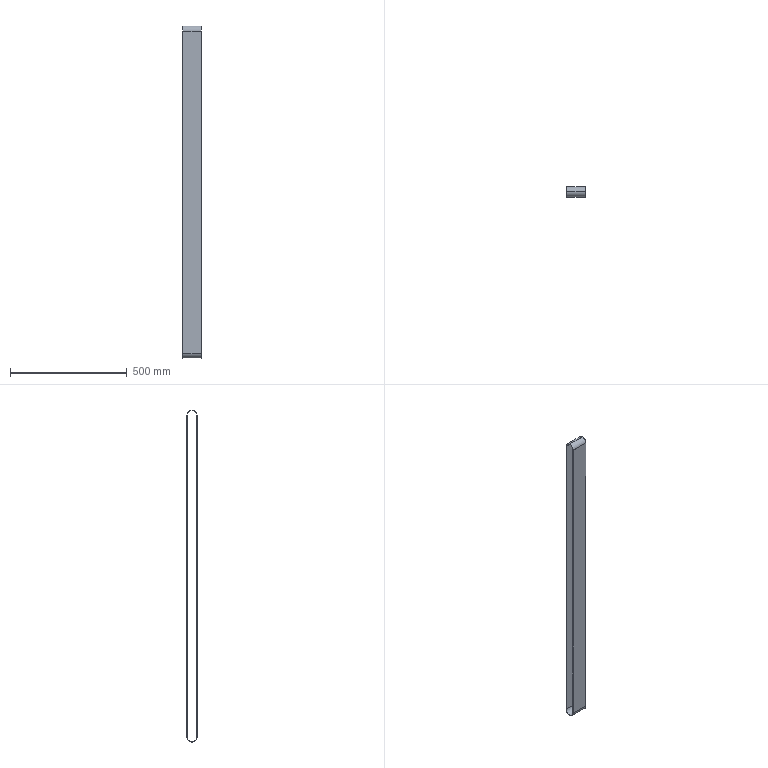Component | SolidWorks | ConveyorBelt-1 | 1 solid | 12 faces | box 78 x 43 x 1423 mm | volume 225572 mm3 | cylinder 6 | plane 6 | commonest cylinder face diameters 41 x3 43 x3
build123d program:
from build123d import *

# Parameters (mm, degrees)
BOSS_EXTRUDE1_DEPTH = 78


with BuildPart() as part:
    # Sketch1 → Boss-Extrude1 (new body)
    with BuildSketch(Plane(origin=(0, 0, 0), x_dir=(0, 0, -1), z_dir=(1, 0, 0))):
        with BuildLine():
            Line((-57.814, 21.5), (1322.186, 21.5))
            ThreePointArc((1322.186, 21.5), (1343.686, 0), (1322.186, -21.5))
            Line((1322.186, -21.5), (-57.814, -21.5))
            ThreePointArc((-57.814, -21.5), (-79.314, 0), (-57.814, 21.5))
        make_face()
        with BuildLine():
            Line((-57.814, 20.5), (1322.186, 20.5))
            ThreePointArc((1322.186, 20.5), (1342.686, 0), (1322.186, -20.5))
            Line((1322.186, -20.5), (-57.814, -20.5))
            ThreePointArc((-57.814, -20.5), (-78.314, 0), (-57.814, 20.5))
        make_face(mode=Mode.SUBTRACT)
    extrude(amount=BOSS_EXTRUDE1_DEPTH)


solid = part.part

# Placed as in the assembly
solid = solid.moved(Location((-44.55, 5.646, 1477.186), (0, 0, 0)))
STEP:
#1=COLOUR_RGB('',0.7922,0.8196,0.9333);
#2=FILL_AREA_STYLE_COLOUR('',#1);
#3=FILL_AREA_STYLE('',(#2));
#4=SURFACE_STYLE_FILL_AREA(#3);
#5=SURFACE_SIDE_STYLE('',(#4));
#6=SURFACE_STYLE_USAGE(.BOTH.,#5);
#7=PRESENTATION_STYLE_ASSIGNMENT((#6));
#8=CARTESIAN_POINT('',(1.317,1.029,60.433));
#9=VERTEX_POINT('',#8);
#10=CARTESIAN_POINT('',(1.317,0.2223,61.24));
#11=VERTEX_POINT('',#10);
#12=CARTESIAN_POINT('',(1.317,0.2223,60.433));
#13=DIRECTION('',(1.,0.,0.));
#14=DIRECTION('',(0.,0.,-1.));
#15=AXIS2_PLACEMENT_3D('',#12,#13,#14);
#16=CIRCLE('',#15,0.8071);
#17=EDGE_CURVE('',#9,#11,#16,.T.);
#18=ORIENTED_EDGE('',*,*,#17,.T.);
#19=CARTESIAN_POINT('',(-1.754,0.2223,61.24));
#20=VERTEX_POINT('',#19);
#21=CARTESIAN_POINT('',(1.317,0.2223,61.24));
#22=DIRECTION('',(-1.,0.,0.));
#23=VECTOR('',#22,39.37);
#24=LINE('',#21,#23);
#25=EDGE_CURVE('',#11,#20,#24,.T.);
#26=ORIENTED_EDGE('',*,*,#25,.T.);
#27=CARTESIAN_POINT('',(-1.754,1.029,60.433));
#28=VERTEX_POINT('',#27);
#29=CARTESIAN_POINT('',(-1.754,0.2223,60.433));
#30=DIRECTION('',(1.,0.,0.));
#31=DIRECTION('',(0.,0.,-1.));
#32=AXIS2_PLACEMENT_3D('',#29,#30,#31);
#33=CIRCLE('',#32,0.8071);
#34=EDGE_CURVE('',#28,#20,#33,.T.);
#35=ORIENTED_EDGE('',*,*,#34,.F.);
#36=CARTESIAN_POINT('',(1.317,1.029,60.433));
#37=DIRECTION('',(-1.,0.,0.));
#38=VECTOR('',#37,39.37);
#39=LINE('',#36,#38);
#40=EDGE_CURVE('',#9,#28,#39,.T.);
#41=ORIENTED_EDGE('',*,*,#40,.F.);
#42=EDGE_LOOP('',(#18,#26,#35,#41));
#43=FACE_OUTER_BOUND('',#42,.T.);
#44=CARTESIAN_POINT('',(1.317,0.2223,60.433));
#45=DIRECTION('',(-1.,0.,0.));
#46=DIRECTION('',(0.,0.,1.));
#47=AXIS2_PLACEMENT_3D('',#44,#45,#46);
#48=CYLINDRICAL_SURFACE('',#47,0.8071);
#49=ADVANCED_FACE('',(#43),#48,.F.);
#50=CARTESIAN_POINT('',(1.317,0.2223,61.28));
#51=VERTEX_POINT('',#50);
#52=CARTESIAN_POINT('',(1.317,-0.6242,60.433));
#53=VERTEX_POINT('',#52);
#54=CARTESIAN_POINT('',(1.317,0.2223,60.433));
#55=DIRECTION('',(1.,0.,0.));
#56=DIRECTION('',(0.,0.,-1.));
#57=AXIS2_PLACEMENT_3D('',#54,#55,#56);
#58=CIRCLE('',#57,0.8465);
#59=EDGE_CURVE('',#51,#53,#58,.T.);
#60=ORIENTED_EDGE('',*,*,#59,.F.);
#61=CARTESIAN_POINT('',(-1.754,0.2223,61.28));
#62=VERTEX_POINT('',#61);
#63=CARTESIAN_POINT('',(1.317,0.2223,61.28));
#64=DIRECTION('',(-1.,0.,0.));
#65=VECTOR('',#64,39.37);
#66=LINE('',#63,#65);
#67=EDGE_CURVE('',#51,#62,#66,.T.);
#68=ORIENTED_EDGE('',*,*,#67,.T.);
#69=CARTESIAN_POINT('',(-1.754,-0.6242,60.433));
#70=VERTEX_POINT('',#69);
#71=CARTESIAN_POINT('',(-1.754,0.2223,60.433));
#72=DIRECTION('',(1.,0.,0.));
#73=DIRECTION('',(0.,0.,-1.));
#74=AXIS2_PLACEMENT_3D('',#71,#72,#73);
#75=CIRCLE('',#74,0.8465);
#76=EDGE_CURVE('',#62,#70,#75,.T.);
#77=ORIENTED_EDGE('',*,*,#76,.T.);
#78=CARTESIAN_POINT('',(1.317,-0.6242,60.433));
#79=DIRECTION('',(-1.,0.,0.));
#80=VECTOR('',#79,39.37);
#81=LINE('',#78,#80);
#82=EDGE_CURVE('',#53,#70,#81,.T.);
#83=ORIENTED_EDGE('',*,*,#82,.F.);
#84=EDGE_LOOP('',(#60,#68,#77,#83));
#85=FACE_OUTER_BOUND('',#84,.T.);
#86=CARTESIAN_POINT('',(1.317,0.2223,60.433));
#87=DIRECTION('',(-1.,0.,0.));
#88=DIRECTION('',(0.,0.,1.));
#89=AXIS2_PLACEMENT_3D('',#86,#87,#88);
#90=CYLINDRICAL_SURFACE('',#89,0.8465);
#91=ADVANCED_FACE('',(#85),#90,.T.);
#92=CARTESIAN_POINT('',(1.317,1.069,60.433));
#93=VERTEX_POINT('',#92);
#94=CARTESIAN_POINT('',(1.317,0.2223,60.433));
#95=DIRECTION('',(1.,0.,0.));
#96=DIRECTION('',(0.,0.,-1.));
#97=AXIS2_PLACEMENT_3D('',#94,#95,#96);
#98=CIRCLE('',#97,0.8465);
#99=EDGE_CURVE('',#93,#51,#98,.T.);
#100=ORIENTED_EDGE('',*,*,#99,.T.);
#101=ORIENTED_EDGE('',*,*,#59,.T.);
#102=CARTESIAN_POINT('',(1.317,-0.6242,6.102));
#103=VERTEX_POINT('',#102);
#104=CARTESIAN_POINT('',(1.317,-0.6242,6.102));
#105=DIRECTION('',(0.,0.,-1.));
#106=VECTOR('',#105,39.37);
#107=LINE('',#104,#106);
#108=EDGE_CURVE('',#53,#103,#107,.T.);
#109=ORIENTED_EDGE('',*,*,#108,.T.);
#110=CARTESIAN_POINT('',(1.317,1.069,6.102));
#111=VERTEX_POINT('',#110);
#112=CARTESIAN_POINT('',(1.317,0.2223,6.102));
#113=DIRECTION('',(1.,0.,0.));
#114=DIRECTION('',(0.,0.,-1.));
#115=AXIS2_PLACEMENT_3D('',#112,#113,#114);
#116=CIRCLE('',#115,0.8465);
#117=EDGE_CURVE('',#103,#111,#116,.T.);
#118=ORIENTED_EDGE('',*,*,#117,.T.);
#119=CARTESIAN_POINT('',(1.317,1.069,60.433));
#120=DIRECTION('',(0.,0.,1.));
#121=VECTOR('',#120,39.37);
#122=LINE('',#119,#121);
#123=EDGE_CURVE('',#111,#93,#122,.T.);
#124=ORIENTED_EDGE('',*,*,#123,.T.);
#125=EDGE_LOOP('',(#100,#101,#109,#118,#124));
#126=FACE_OUTER_BOUND('',#125,.T.);
#127=CARTESIAN_POINT('',(1.317,-0.5848,60.433));
#128=VERTEX_POINT('',#127);
#129=CARTESIAN_POINT('',(1.317,-0.5848,6.102));
#130=VERTEX_POINT('',#129);
#131=CARTESIAN_POINT('',(1.317,-0.5848,6.102));
#132=DIRECTION('',(0.,0.,-1.));
#133=VECTOR('',#132,39.37);
#134=LINE('',#131,#133);
#135=EDGE_CURVE('',#128,#130,#134,.T.);
#136=ORIENTED_EDGE('',*,*,#135,.F.);
#137=CARTESIAN_POINT('',(1.317,0.2223,60.433));
#138=DIRECTION('',(1.,0.,0.));
#139=DIRECTION('',(0.,0.,-1.));
#140=AXIS2_PLACEMENT_3D('',#137,#138,#139);
#141=CIRCLE('',#140,0.8071);
#142=EDGE_CURVE('',#11,#128,#141,.T.);
#143=ORIENTED_EDGE('',*,*,#142,.F.);
#144=ORIENTED_EDGE('',*,*,#17,.F.);
#145=CARTESIAN_POINT('',(1.317,1.029,6.102));
#146=VERTEX_POINT('',#145);
#147=CARTESIAN_POINT('',(1.317,1.029,60.433));
#148=DIRECTION('',(0.,0.,1.));
#149=VECTOR('',#148,39.37);
#150=LINE('',#147,#149);
#151=EDGE_CURVE('',#146,#9,#150,.T.);
#152=ORIENTED_EDGE('',*,*,#151,.F.);
#153=CARTESIAN_POINT('',(1.317,0.2223,6.102));
#154=DIRECTION('',(1.,0.,0.));
#155=DIRECTION('',(0.,0.,-1.));
#156=AXIS2_PLACEMENT_3D('',#153,#154,#155);
#157=CIRCLE('',#156,0.8071);
#158=EDGE_CURVE('',#130,#146,#157,.T.);
#159=ORIENTED_EDGE('',*,*,#158,.F.);
#160=EDGE_LOOP('',(#136,#143,#144,#152,#159));
#161=FACE_BOUND('',#160,.T.);
#162=CARTESIAN_POINT('',(1.317,0.2223,60.433));
#163=DIRECTION('',(1.,0.,0.));
#164=DIRECTION('',(0.,0.,-1.));
#165=AXIS2_PLACEMENT_3D('',#162,#163,#164);
#166=PLANE('',#165);
#167=ADVANCED_FACE('',(#126,#161),#166,.T.);
#168=CARTESIAN_POINT('',(-1.754,1.069,60.433));
#169=VERTEX_POINT('',#168);
#170=CARTESIAN_POINT('',(-1.754,0.2223,60.433));
#171=DIRECTION('',(1.,0.,0.));
#172=DIRECTION('',(0.,0.,-1.));
#173=AXIS2_PLACEMENT_3D('',#170,#171,#172);
#174=CIRCLE('',#173,0.8465);
#175=EDGE_CURVE('',#169,#62,#174,.T.);
#176=ORIENTED_EDGE('',*,*,#175,.F.);
#177=CARTESIAN_POINT('',(-1.754,1.069,6.102));
#178=VERTEX_POINT('',#177);
#179=CARTESIAN_POINT('',(-1.754,1.069,60.433));
#180=DIRECTION('',(0.,0.,1.));
#181=VECTOR('',#180,39.37);
#182=LINE('',#179,#181);
#183=EDGE_CURVE('',#178,#169,#182,.T.);
#184=ORIENTED_EDGE('',*,*,#183,.F.);
#185=CARTESIAN_POINT('',(-1.754,-0.6242,6.102));
#186=VERTEX_POINT('',#185);
#187=CARTESIAN_POINT('',(-1.754,0.2223,6.102));
#188=DIRECTION('',(1.,0.,0.));
#189=DIRECTION('',(0.,0.,-1.));
#190=AXIS2_PLACEMENT_3D('',#187,#188,#189);
#191=CIRCLE('',#190,0.8465);
#192=EDGE_CURVE('',#186,#178,#191,.T.);
#193=ORIENTED_EDGE('',*,*,#192,.F.);
#194=CARTESIAN_POINT('',(-1.754,-0.6242,6.102));
#195=DIRECTION('',(0.,0.,-1.));
#196=VECTOR('',#195,39.37);
#197=LINE('',#194,#196);
#198=EDGE_CURVE('',#70,#186,#197,.T.);
#199=ORIENTED_EDGE('',*,*,#198,.F.);
#200=ORIENTED_EDGE('',*,*,#76,.F.);
#201=EDGE_LOOP('',(#176,#184,#193,#199,#200));
#202=FACE_OUTER_BOUND('',#201,.T.);
#203=ORIENTED_EDGE('',*,*,#34,.T.);
#204=CARTESIAN_POINT('',(-1.754,-0.5848,60.433));
#205=VERTEX_POINT('',#204);
#206=CARTESIAN_POINT('',(-1.754,0.2223,60.433));
#207=DIRECTION('',(1.,0.,0.));
#208=DIRECTION('',(0.,0.,-1.));
#209=AXIS2_PLACEMENT_3D('',#206,#207,#208);
#210=CIRCLE('',#209,0.8071);
#211=EDGE_CURVE('',#20,#205,#210,.T.);
#212=ORIENTED_EDGE('',*,*,#211,.T.);
#213=CARTESIAN_POINT('',(-1.754,-0.5848,6.102));
#214=VERTEX_POINT('',#213);
#215=CARTESIAN_POINT('',(-1.754,-0.5848,6.102));
#216=DIRECTION('',(0.,0.,-1.));
#217=VECTOR('',#216,39.37);
#218=LINE('',#215,#217);
#219=EDGE_CURVE('',#205,#214,#218,.T.);
#220=ORIENTED_EDGE('',*,*,#219,.T.);
#221=CARTESIAN_POINT('',(-1.754,1.029,6.102));
#222=VERTEX_POINT('',#221);
#223=CARTESIAN_POINT('',(-1.754,0.2223,6.102));
#224=DIRECTION('',(1.,0.,0.));
#225=DIRECTION('',(0.,0.,-1.));
#226=AXIS2_PLACEMENT_3D('',#223,#224,#225);
#227=CIRCLE('',#226,0.8071);
#228=EDGE_CURVE('',#214,#222,#227,.T.);
#229=ORIENTED_EDGE('',*,*,#228,.T.);
#230=CARTESIAN_POINT('',(-1.754,1.029,60.433));
#231=DIRECTION('',(0.,0.,1.));
#232=VECTOR('',#231,39.37);
#233=LINE('',#230,#232);
#234=EDGE_CURVE('',#222,#28,#233,.T.);
#235=ORIENTED_EDGE('',*,*,#234,.T.);
#236=EDGE_LOOP('',(#203,#212,#220,#229,#235));
#237=FACE_BOUND('',#236,.T.);
#238=CARTESIAN_POINT('',(-1.754,0.2223,60.433));
#239=DIRECTION('',(1.,0.,0.));
#240=DIRECTION('',(0.,0.,-1.));
#241=AXIS2_PLACEMENT_3D('',#238,#239,#240);
#242=PLANE('',#241);
#243=ADVANCED_FACE('',(#202,#237),#242,.F.);
#244=ORIENTED_EDGE('',*,*,#67,.F.);
#245=ORIENTED_EDGE('',*,*,#99,.F.);
#246=CARTESIAN_POINT('',(1.317,1.069,60.433));
#247=DIRECTION('',(-1.,0.,0.));
#248=VECTOR('',#247,39.37);
#249=LINE('',#246,#248);
#250=EDGE_CURVE('',#93,#169,#249,.T.);
#251=ORIENTED_EDGE('',*,*,#250,.T.);
#252=ORIENTED_EDGE('',*,*,#175,.T.);
#253=EDGE_LOOP('',(#244,#245,#251,#252));
#254=FACE_OUTER_BOUND('',#253,.T.);
#255=CARTESIAN_POINT('',(1.317,0.2223,60.433));
#256=DIRECTION('',(-1.,0.,0.));
#257=DIRECTION('',(0.,0.,1.));
#258=AXIS2_PLACEMENT_3D('',#255,#256,#257);
#259=CYLINDRICAL_SURFACE('',#258,0.8465);
#260=ADVANCED_FACE('',(#254),#259,.T.);
#261=ORIENTED_EDGE('',*,*,#198,.T.);
#262=CARTESIAN_POINT('',(1.317,-0.6242,6.102));
#263=DIRECTION('',(-1.,0.,0.));
#264=VECTOR('',#263,39.37);
#265=LINE('',#262,#264);
#266=EDGE_CURVE('',#103,#186,#265,.T.);
#267=ORIENTED_EDGE('',*,*,#266,.F.);
#268=ORIENTED_EDGE('',*,*,#108,.F.);
#269=ORIENTED_EDGE('',*,*,#82,.T.);
#270=EDGE_LOOP('',(#261,#267,#268,#269));
#271=FACE_OUTER_BOUND('',#270,.T.);
#272=CARTESIAN_POINT('',(1.317,-0.6242,6.102));
#273=DIRECTION('',(0.,1.,0.));
#274=DIRECTION('',(0.,-0.,1.));
#275=AXIS2_PLACEMENT_3D('',#272,#273,#274);
#276=PLANE('',#275);
#277=ADVANCED_FACE('',(#271),#276,.F.);
#278=ORIENTED_EDGE('',*,*,#192,.T.);
#279=CARTESIAN_POINT('',(1.317,1.069,6.102));
#280=DIRECTION('',(-1.,0.,0.));
#281=VECTOR('',#280,39.37);
#282=LINE('',#279,#281);
#283=EDGE_CURVE('',#111,#178,#282,.T.);
#284=ORIENTED_EDGE('',*,*,#283,.F.);
#285=ORIENTED_EDGE('',*,*,#117,.F.);
#286=ORIENTED_EDGE('',*,*,#266,.T.);
#287=EDGE_LOOP('',(#278,#284,#285,#286));
#288=FACE_OUTER_BOUND('',#287,.T.);
#289=CARTESIAN_POINT('',(1.317,0.2223,6.102));
#290=DIRECTION('',(-1.,0.,0.));
#291=DIRECTION('',(0.,0.,1.));
#292=AXIS2_PLACEMENT_3D('',#289,#290,#291);
#293=CYLINDRICAL_SURFACE('',#292,0.8465);
#294=ADVANCED_FACE('',(#288),#293,.T.);
#295=ORIENTED_EDGE('',*,*,#183,.T.);
#296=ORIENTED_EDGE('',*,*,#250,.F.);
#297=ORIENTED_EDGE('',*,*,#123,.F.);
#298=ORIENTED_EDGE('',*,*,#283,.T.);
#299=EDGE_LOOP('',(#295,#296,#297,#298));
#300=FACE_OUTER_BOUND('',#299,.T.);
#301=CARTESIAN_POINT('',(1.317,1.069,60.433));
#302=DIRECTION('',(0.,-1.,0.));
#303=DIRECTION('',(0.,0.,-1.));
#304=AXIS2_PLACEMENT_3D('',#301,#302,#303);
#305=PLANE('',#304);
#306=ADVANCED_FACE('',(#300),#305,.F.);
#307=ORIENTED_EDGE('',*,*,#25,.F.);
#308=ORIENTED_EDGE('',*,*,#142,.T.);
#309=CARTESIAN_POINT('',(1.317,-0.5848,60.433));
#310=DIRECTION('',(-1.,0.,0.));
#311=VECTOR('',#310,39.37);
#312=LINE('',#309,#311);
#313=EDGE_CURVE('',#128,#205,#312,.T.);
#314=ORIENTED_EDGE('',*,*,#313,.T.);
#315=ORIENTED_EDGE('',*,*,#211,.F.);
#316=EDGE_LOOP('',(#307,#308,#314,#315));
#317=FACE_OUTER_BOUND('',#316,.T.);
#318=CARTESIAN_POINT('',(1.317,0.2223,60.433));
#319=DIRECTION('',(-1.,0.,0.));
#320=DIRECTION('',(0.,0.,1.));
#321=AXIS2_PLACEMENT_3D('',#318,#319,#320);
#322=CYLINDRICAL_SURFACE('',#321,0.8071);
#323=ADVANCED_FACE('',(#317),#322,.F.);
#324=ORIENTED_EDGE('',*,*,#219,.F.);
#325=ORIENTED_EDGE('',*,*,#313,.F.);
#326=ORIENTED_EDGE('',*,*,#135,.T.);
#327=CARTESIAN_POINT('',(1.317,-0.5848,6.102));
#328=DIRECTION('',(-1.,0.,0.));
#329=VECTOR('',#328,39.37);
#330=LINE('',#327,#329);
#331=EDGE_CURVE('',#130,#214,#330,.T.);
#332=ORIENTED_EDGE('',*,*,#331,.T.);
#333=EDGE_LOOP('',(#324,#325,#326,#332));
#334=FACE_OUTER_BOUND('',#333,.T.);
#335=CARTESIAN_POINT('',(1.317,-0.5848,6.102));
#336=DIRECTION('',(0.,1.,0.));
#337=DIRECTION('',(0.,0.,1.));
#338=AXIS2_PLACEMENT_3D('',#335,#336,#337);
#339=PLANE('',#338);
#340=ADVANCED_FACE('',(#334),#339,.T.);
#341=ORIENTED_EDGE('',*,*,#228,.F.);
#342=ORIENTED_EDGE('',*,*,#331,.F.);
#343=ORIENTED_EDGE('',*,*,#158,.T.);
#344=CARTESIAN_POINT('',(1.317,1.029,6.102));
#345=DIRECTION('',(-1.,0.,0.));
#346=VECTOR('',#345,39.37);
#347=LINE('',#344,#346);
#348=EDGE_CURVE('',#146,#222,#347,.T.);
#349=ORIENTED_EDGE('',*,*,#348,.T.);
#350=EDGE_LOOP('',(#341,#342,#343,#349));
#351=FACE_OUTER_BOUND('',#350,.T.);
#352=CARTESIAN_POINT('',(1.317,0.2223,6.102));
#353=DIRECTION('',(-1.,0.,0.));
#354=DIRECTION('',(0.,0.,1.));
#355=AXIS2_PLACEMENT_3D('',#352,#353,#354);
#356=CYLINDRICAL_SURFACE('',#355,0.8071);
#357=ADVANCED_FACE('',(#351),#356,.F.);
#358=ORIENTED_EDGE('',*,*,#234,.F.);
#359=ORIENTED_EDGE('',*,*,#348,.F.);
#360=ORIENTED_EDGE('',*,*,#151,.T.);
#361=ORIENTED_EDGE('',*,*,#40,.T.);
#362=EDGE_LOOP('',(#358,#359,#360,#361));
#363=FACE_OUTER_BOUND('',#362,.T.);
#364=CARTESIAN_POINT('',(1.317,1.029,60.433));
#365=DIRECTION('',(0.,-1.,0.));
#366=DIRECTION('',(0.,0.,-1.));
#367=AXIS2_PLACEMENT_3D('',#364,#365,#366);
#368=PLANE('',#367);
#369=ADVANCED_FACE('',(#363),#368,.T.);
#370=CLOSED_SHELL('',(#49,#91,#167,#243,#260,#277,#294,#306,#323,#340,#357,#369));
#371=MANIFOLD_SOLID_BREP('',#370);
#372=STYLED_ITEM('',(#7),#371);
#373=(LENGTH_UNIT()NAMED_UNIT(*)SI_UNIT($,.METRE.));
#374=LENGTH_MEASURE_WITH_UNIT(LENGTH_MEASURE(0.0254),#373);
#375=DIMENSIONAL_EXPONENTS(1.,0.,0.,0.,0.,0.,0.);
#376=(CONVERSION_BASED_UNIT('',#374)LENGTH_UNIT()NAMED_UNIT(#375));
#377=UNCERTAINTY_MEASURE_WITH_UNIT(LENGTH_MEASURE(0.00001),#376,'','');
#378=(NAMED_UNIT(*)PLANE_ANGLE_UNIT()SI_UNIT($,.RADIAN.));
#379=(NAMED_UNIT(*)SI_UNIT($,.STERADIAN.)SOLID_ANGLE_UNIT());
#380=(GEOMETRIC_REPRESENTATION_CONTEXT(3)GLOBAL_UNCERTAINTY_ASSIGNED_CONTEXT((#377))GLOBAL_UNIT_ASSIGNED_CONTEXT((#376,#378,#379))REPRESENTATION_CONTEXT('',''));
#381=MECHANICAL_DESIGN_GEOMETRIC_PRESENTATION_REPRESENTATION('',(#372),#380);
#382=CARTESIAN_POINT('',(0.,0.,0.));
#383=DIRECTION('',(0.,0.,1.));
#384=DIRECTION('',(1.,0.,0.));
#385=AXIS2_PLACEMENT_3D('',#382,#383,#384);
#386=(LENGTH_UNIT()NAMED_UNIT(*)SI_UNIT($,.METRE.));
#387=LENGTH_MEASURE_WITH_UNIT(LENGTH_MEASURE(0.0254),#386);
#388=DIMENSIONAL_EXPONENTS(1.,0.,0.,0.,0.,0.,0.);
#389=(CONVERSION_BASED_UNIT('',#387)LENGTH_UNIT()NAMED_UNIT(#388));
#390=UNCERTAINTY_MEASURE_WITH_UNIT(LENGTH_MEASURE(0.00001),#389,'','');
#391=(NAMED_UNIT(*)PLANE_ANGLE_UNIT()SI_UNIT($,.RADIAN.));
#392=(NAMED_UNIT(*)SI_UNIT($,.STERADIAN.)SOLID_ANGLE_UNIT());
#393=(GEOMETRIC_REPRESENTATION_CONTEXT(3)GLOBAL_UNCERTAINTY_ASSIGNED_CONTEXT((#390))GLOBAL_UNIT_ASSIGNED_CONTEXT((#389,#391,#392))REPRESENTATION_CONTEXT('',''));
#394=ADVANCED_BREP_SHAPE_REPRESENTATION('',(#371,#385),#393);
#395=PRESENTATION_LAYER_ASSIGNMENT('','',(#372));